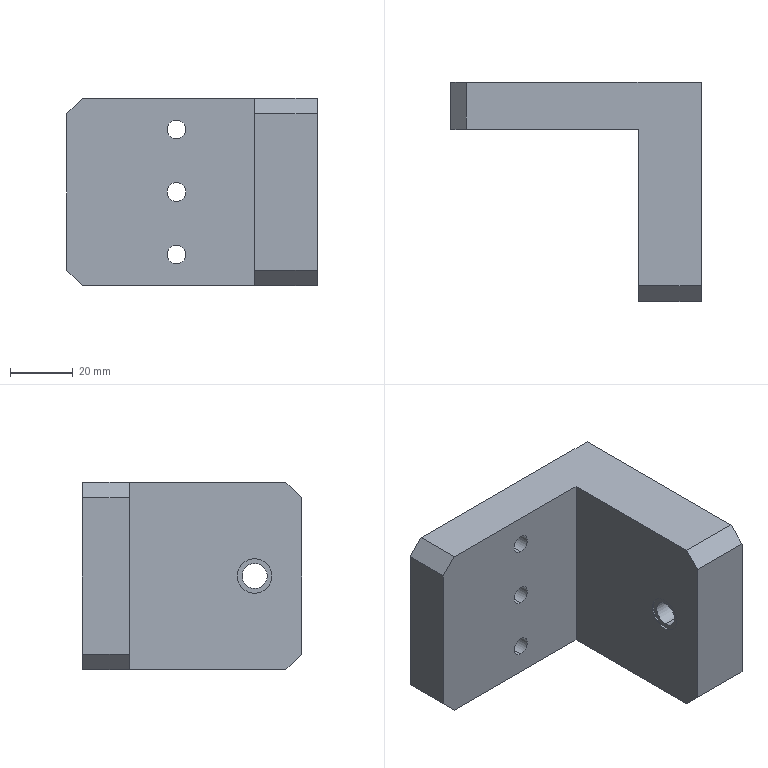Component | SolidWorks | ElectricalBoxAssembly2-1_AuxiliaryWheelFrame-1 | 1 solid | 23 faces | box 80 x 70 x 60 mm | volume 134825 mm3 | plane 13 | cylinder 10 | commonest cylinder face diameters 6 x6 11 x2 8 x2
build123d program:
from build123d import *

# Parameters (mm, degrees)
BOSS_EXTRUDE1_DEPTH           = 30
M8_TAPPED_HOLE1_D             = 8
SKETCH5_R                     = 2
CUT_EXTRUDE1_DEPTH            = 102.612
CHAMFER1_SIZE                 = 5
M6_TAPPED_HOLE2_D             = 6
M6_TAPPED_HOLE3_D             = 6
SKETCH1_R                     = 5.5
M8_SHOULDERSEAT_D11X0_5_DEPTH = 0.5


with BuildPart() as part:
    # Sketch1_2 → Boss-Extrude1 (new, symmetric)
    with BuildSketch(Plane.XY):
        Polygon((0, 0), (0, 70), (20, 70), (20, 15), (80, 15), (80, 0), align=None)
    extrude(amount=BOSS_EXTRUDE1_DEPTH, both=True)

    # M8 Tapped Hole1 (through all)
    with Locations(Plane(origin=(20, 0, 0), x_dir=(0, 0, -1), z_dir=(1, 0, 0))):
        with Locations((0, 55)):
            Hole(M8_TAPPED_HOLE1_D / 2)

    # Sketch5 → Cut-Extrude1 (cut, through all)
    with BuildSketch(Plane(origin=(0, 15, 0), x_dir=(1, 0, 0), z_dir=(0, 1, 0))):
        with Locations(Location((45, 20, 0), (0, 0, 270))):
            Circle(SKETCH5_R)
        with Locations(Location((45, -20, 0), (0, 0, 270))):
            Circle(SKETCH5_R)
        with Locations(Location((45, 0, 0), (0, 0, 270))):
            Circle(SKETCH5_R)
    extrude(amount=-CUT_EXTRUDE1_DEPTH, mode=Mode.SUBTRACT)

    # Chamfer1
    chamfer1_edges = [part.edges().sort_by_distance(p)[0] for p in [
        (10, 70, 30),
        (10, 70, -30),
        (80, 7.5, 30),
        (80, 7.5, -30),
    ]]
    chamfer(chamfer1_edges, length=CHAMFER1_SIZE)

    # M6 Tapped Hole2 (through all)
    with Locations(Plane(origin=(0, 15, 0), x_dir=(1, 0, 0), z_dir=(0, 1, 0))):
        with Locations((45, 20), (45, -20)):
            Hole(M6_TAPPED_HOLE2_D / 2)

    # M6 Tapped Hole3 (through all)
    with Locations(Plane(origin=(0, 15, 0), x_dir=(1, 0, 0), z_dir=(0, 1, 0))):
        with Locations((45, 0)):
            Hole(M6_TAPPED_HOLE3_D / 2)

    # Sketch1 → M8_ShoulderSeat_D11x0.5 (cut)
    with BuildSketch(Plane(origin=(20, 0, 0), x_dir=(0, 0, -1), z_dir=(1, 0, 0))):
        with Locations(Location((0, 55, 0), (0, 0, 90))):
            Circle(SKETCH1_R)
    extrude(amount=-M8_SHOULDERSEAT_D11X0_5_DEPTH, mode=Mode.SUBTRACT)


solid = part.part

# Placed as in the assembly
solid = solid.moved(Location((755.468, 389.666, 1526.399), (0, 0, 180)))
STEP:
#1=CARTESIAN_POINT('',(28.975,13.392,60.094));
#2=VERTEX_POINT('',#1);
#3=CARTESIAN_POINT('',(28.975,12.959,60.094));
#4=VERTEX_POINT('',#3);
#5=CARTESIAN_POINT('',(28.975,13.176,60.094));
#6=DIRECTION('',(-1.,-0.,-0.));
#7=DIRECTION('',(0.,-1.,0.));
#8=AXIS2_PLACEMENT_3D('',#5,#6,#7);
#9=CIRCLE('',#8,0.2165);
#10=EDGE_CURVE('',#2,#4,#9,.T.);
#11=ORIENTED_EDGE('',*,*,#10,.F.);
#12=CARTESIAN_POINT('',(28.955,13.392,60.094));
#13=VERTEX_POINT('',#12);
#14=CARTESIAN_POINT('',(28.975,13.392,60.094));
#15=DIRECTION('',(-1.,-0.,-0.));
#16=VECTOR('',#15,39.37);
#17=LINE('',#14,#16);
#18=EDGE_CURVE('',#2,#13,#17,.T.);
#19=ORIENTED_EDGE('',*,*,#18,.T.);
#20=CARTESIAN_POINT('',(28.955,12.959,60.094));
#21=VERTEX_POINT('',#20);
#22=CARTESIAN_POINT('',(28.955,13.176,60.094));
#23=DIRECTION('',(-1.,-0.,-0.));
#24=DIRECTION('',(0.,-1.,0.));
#25=AXIS2_PLACEMENT_3D('',#22,#23,#24);
#26=CIRCLE('',#25,0.2165);
#27=EDGE_CURVE('',#13,#21,#26,.T.);
#28=ORIENTED_EDGE('',*,*,#27,.T.);
#29=CARTESIAN_POINT('',(28.975,12.959,60.094));
#30=DIRECTION('',(-1.,-0.,-0.));
#31=VECTOR('',#30,39.37);
#32=LINE('',#29,#31);
#33=EDGE_CURVE('',#4,#21,#32,.T.);
#34=ORIENTED_EDGE('',*,*,#33,.F.);
#35=EDGE_LOOP('',(#11,#19,#28,#34));
#36=FACE_OUTER_BOUND('',#35,.T.);
#37=CARTESIAN_POINT('',(28.975,13.176,60.094));
#38=DIRECTION('',(-1.,-0.,-0.));
#39=DIRECTION('',(0.,-1.,0.));
#40=AXIS2_PLACEMENT_3D('',#37,#38,#39);
#41=CYLINDRICAL_SURFACE('',#40,0.2165);
#42=ADVANCED_FACE('',(#36),#41,.F.);
#43=CARTESIAN_POINT('',(27.971,15.341,59.976));
#44=VERTEX_POINT('',#43);
#45=CARTESIAN_POINT('',(27.971,15.341,60.213));
#46=VERTEX_POINT('',#45);
#47=CARTESIAN_POINT('',(27.971,15.341,60.094));
#48=DIRECTION('',(0.,-1.,-0.));
#49=DIRECTION('',(0.,0.,1.));
#50=AXIS2_PLACEMENT_3D('',#47,#48,#49);
#51=CIRCLE('',#50,0.1181);
#52=EDGE_CURVE('',#44,#46,#51,.T.);
#53=ORIENTED_EDGE('',*,*,#52,.F.);
#54=CARTESIAN_POINT('',(27.971,14.751,59.976));
#55=VERTEX_POINT('',#54);
#56=CARTESIAN_POINT('',(27.971,14.751,59.976));
#57=DIRECTION('',(0.,-1.,-0.));
#58=VECTOR('',#57,39.37);
#59=LINE('',#56,#58);
#60=EDGE_CURVE('',#44,#55,#59,.T.);
#61=ORIENTED_EDGE('',*,*,#60,.T.);
#62=CARTESIAN_POINT('',(27.971,14.751,60.213));
#63=VERTEX_POINT('',#62);
#64=CARTESIAN_POINT('',(27.971,14.751,60.094));
#65=DIRECTION('',(0.,-1.,-0.));
#66=DIRECTION('',(0.,0.,1.));
#67=AXIS2_PLACEMENT_3D('',#64,#65,#66);
#68=CIRCLE('',#67,0.1181);
#69=EDGE_CURVE('',#55,#63,#68,.T.);
#70=ORIENTED_EDGE('',*,*,#69,.T.);
#71=CARTESIAN_POINT('',(27.971,14.751,60.213));
#72=DIRECTION('',(0.,-1.,-0.));
#73=VECTOR('',#72,39.37);
#74=LINE('',#71,#73);
#75=EDGE_CURVE('',#46,#63,#74,.T.);
#76=ORIENTED_EDGE('',*,*,#75,.F.);
#77=EDGE_LOOP('',(#53,#61,#70,#76));
#78=FACE_OUTER_BOUND('',#77,.T.);
#79=CARTESIAN_POINT('',(27.971,14.751,60.094));
#80=DIRECTION('',(0.,-1.,-0.));
#81=DIRECTION('',(0.,0.,1.));
#82=AXIS2_PLACEMENT_3D('',#79,#80,#81);
#83=CYLINDRICAL_SURFACE('',#82,0.1181);
#84=ADVANCED_FACE('',(#78),#83,.F.);
#85=CARTESIAN_POINT('',(27.971,15.341,59.189));
#86=VERTEX_POINT('',#85);
#87=CARTESIAN_POINT('',(27.971,15.341,59.425));
#88=VERTEX_POINT('',#87);
#89=CARTESIAN_POINT('',(27.971,15.341,59.307));
#90=DIRECTION('',(0.,-1.,-0.));
#91=DIRECTION('',(0.,0.,1.));
#92=AXIS2_PLACEMENT_3D('',#89,#90,#91);
#93=CIRCLE('',#92,0.1181);
#94=EDGE_CURVE('',#86,#88,#93,.T.);
#95=ORIENTED_EDGE('',*,*,#94,.F.);
#96=CARTESIAN_POINT('',(27.971,14.751,59.189));
#97=VERTEX_POINT('',#96);
#98=CARTESIAN_POINT('',(27.971,14.751,59.189));
#99=DIRECTION('',(0.,-1.,-0.));
#100=VECTOR('',#99,39.37);
#101=LINE('',#98,#100);
#102=EDGE_CURVE('',#86,#97,#101,.T.);
#103=ORIENTED_EDGE('',*,*,#102,.T.);
#104=CARTESIAN_POINT('',(27.971,14.751,59.425));
#105=VERTEX_POINT('',#104);
#106=CARTESIAN_POINT('',(27.971,14.751,59.307));
#107=DIRECTION('',(0.,-1.,-0.));
#108=DIRECTION('',(0.,0.,1.));
#109=AXIS2_PLACEMENT_3D('',#106,#107,#108);
#110=CIRCLE('',#109,0.1181);
#111=EDGE_CURVE('',#97,#105,#110,.T.);
#112=ORIENTED_EDGE('',*,*,#111,.T.);
#113=CARTESIAN_POINT('',(27.971,14.751,59.425));
#114=DIRECTION('',(0.,-1.,-0.));
#115=VECTOR('',#114,39.37);
#116=LINE('',#113,#115);
#117=EDGE_CURVE('',#88,#105,#116,.T.);
#118=ORIENTED_EDGE('',*,*,#117,.F.);
#119=EDGE_LOOP('',(#95,#103,#112,#118));
#120=FACE_OUTER_BOUND('',#119,.T.);
#121=CARTESIAN_POINT('',(27.971,14.751,59.307));
#122=DIRECTION('',(0.,-1.,-0.));
#123=DIRECTION('',(0.,0.,1.));
#124=AXIS2_PLACEMENT_3D('',#121,#122,#123);
#125=CYLINDRICAL_SURFACE('',#124,0.1181);
#126=ADVANCED_FACE('',(#120),#125,.F.);
#127=CARTESIAN_POINT('',(27.971,15.341,60.764));
#128=VERTEX_POINT('',#127);
#129=CARTESIAN_POINT('',(27.971,15.341,61.));
#130=VERTEX_POINT('',#129);
#131=CARTESIAN_POINT('',(27.971,15.341,60.882));
#132=DIRECTION('',(0.,-1.,-0.));
#133=DIRECTION('',(0.,0.,1.));
#134=AXIS2_PLACEMENT_3D('',#131,#132,#133);
#135=CIRCLE('',#134,0.1181);
#136=EDGE_CURVE('',#128,#130,#135,.T.);
#137=ORIENTED_EDGE('',*,*,#136,.F.);
#138=CARTESIAN_POINT('',(27.971,14.751,60.764));
#139=VERTEX_POINT('',#138);
#140=CARTESIAN_POINT('',(27.971,14.751,60.764));
#141=DIRECTION('',(0.,-1.,-0.));
#142=VECTOR('',#141,39.37);
#143=LINE('',#140,#142);
#144=EDGE_CURVE('',#128,#139,#143,.T.);
#145=ORIENTED_EDGE('',*,*,#144,.T.);
#146=CARTESIAN_POINT('',(27.971,14.751,61.));
#147=VERTEX_POINT('',#146);
#148=CARTESIAN_POINT('',(27.971,14.751,60.882));
#149=DIRECTION('',(0.,-1.,-0.));
#150=DIRECTION('',(0.,0.,1.));
#151=AXIS2_PLACEMENT_3D('',#148,#149,#150);
#152=CIRCLE('',#151,0.1181);
#153=EDGE_CURVE('',#139,#147,#152,.T.);
#154=ORIENTED_EDGE('',*,*,#153,.T.);
#155=CARTESIAN_POINT('',(27.971,14.751,61.));
#156=DIRECTION('',(0.,-1.,-0.));
#157=VECTOR('',#156,39.37);
#158=LINE('',#155,#157);
#159=EDGE_CURVE('',#130,#147,#158,.T.);
#160=ORIENTED_EDGE('',*,*,#159,.F.);
#161=EDGE_LOOP('',(#137,#145,#154,#160));
#162=FACE_OUTER_BOUND('',#161,.T.);
#163=CARTESIAN_POINT('',(27.971,14.751,60.882));
#164=DIRECTION('',(0.,-1.,-0.));
#165=DIRECTION('',(0.,0.,1.));
#166=AXIS2_PLACEMENT_3D('',#163,#164,#165);
#167=CYLINDRICAL_SURFACE('',#166,0.1181);
#168=ADVANCED_FACE('',(#162),#167,.F.);
#169=CARTESIAN_POINT('',(29.743,13.176,60.252));
#170=VERTEX_POINT('',#169);
#171=CARTESIAN_POINT('',(29.743,13.176,59.937));
#172=VERTEX_POINT('',#171);
#173=CARTESIAN_POINT('',(29.743,13.176,60.094));
#174=DIRECTION('',(-1.,-0.,-0.));
#175=DIRECTION('',(0.,0.,-1.));
#176=AXIS2_PLACEMENT_3D('',#173,#174,#175);
#177=CIRCLE('',#176,0.1575);
#178=EDGE_CURVE('',#170,#172,#177,.T.);
#179=ORIENTED_EDGE('',*,*,#178,.F.);
#180=CARTESIAN_POINT('',(28.975,13.176,60.252));
#181=VERTEX_POINT('',#180);
#182=CARTESIAN_POINT('',(28.955,13.176,60.252));
#183=DIRECTION('',(-1.,-0.,-0.));
#184=VECTOR('',#183,39.37);
#185=LINE('',#182,#184);
#186=EDGE_CURVE('',#170,#181,#185,.T.);
#187=ORIENTED_EDGE('',*,*,#186,.T.);
#188=CARTESIAN_POINT('',(28.975,13.176,59.937));
#189=VERTEX_POINT('',#188);
#190=CARTESIAN_POINT('',(28.975,13.176,60.094));
#191=DIRECTION('',(1.,0.,0.));
#192=DIRECTION('',(0.,-1.,0.));
#193=AXIS2_PLACEMENT_3D('',#190,#191,#192);
#194=CIRCLE('',#193,0.1575);
#195=EDGE_CURVE('',#189,#181,#194,.T.);
#196=ORIENTED_EDGE('',*,*,#195,.F.);
#197=CARTESIAN_POINT('',(28.955,13.176,59.937));
#198=DIRECTION('',(-1.,-0.,-0.));
#199=VECTOR('',#198,39.37);
#200=LINE('',#197,#199);
#201=EDGE_CURVE('',#172,#189,#200,.T.);
#202=ORIENTED_EDGE('',*,*,#201,.F.);
#203=EDGE_LOOP('',(#179,#187,#196,#202));
#204=FACE_OUTER_BOUND('',#203,.T.);
#205=CARTESIAN_POINT('',(28.955,13.176,60.094));
#206=DIRECTION('',(-1.,-0.,-0.));
#207=DIRECTION('',(0.,0.,-1.));
#208=AXIS2_PLACEMENT_3D('',#205,#206,#207);
#209=CYLINDRICAL_SURFACE('',#208,0.1575);
#210=ADVANCED_FACE('',(#204),#209,.F.);
#211=ORIENTED_EDGE('',*,*,#186,.F.);
#212=CARTESIAN_POINT('',(29.743,13.176,60.094));
#213=DIRECTION('',(-1.,-0.,-0.));
#214=DIRECTION('',(0.,0.,-1.));
#215=AXIS2_PLACEMENT_3D('',#212,#213,#214);
#216=CIRCLE('',#215,0.1575);
#217=EDGE_CURVE('',#172,#170,#216,.T.);
#218=ORIENTED_EDGE('',*,*,#217,.F.);
#219=ORIENTED_EDGE('',*,*,#201,.T.);
#220=CARTESIAN_POINT('',(28.975,13.176,60.094));
#221=DIRECTION('',(1.,0.,0.));
#222=DIRECTION('',(0.,-1.,0.));
#223=AXIS2_PLACEMENT_3D('',#220,#221,#222);
#224=CIRCLE('',#223,0.1575);
#225=EDGE_CURVE('',#181,#189,#224,.T.);
#226=ORIENTED_EDGE('',*,*,#225,.F.);
#227=EDGE_LOOP('',(#211,#218,#219,#226));
#228=FACE_OUTER_BOUND('',#227,.T.);
#229=CARTESIAN_POINT('',(28.955,13.176,60.094));
#230=DIRECTION('',(-1.,-0.,-0.));
#231=DIRECTION('',(0.,0.,-1.));
#232=AXIS2_PLACEMENT_3D('',#229,#230,#231);
#233=CYLINDRICAL_SURFACE('',#232,0.1575);
#234=ADVANCED_FACE('',(#228),#233,.F.);
#235=CARTESIAN_POINT('',(27.971,15.341,60.094));
#236=DIRECTION('',(0.,-1.,-0.));
#237=DIRECTION('',(0.,0.,1.));
#238=AXIS2_PLACEMENT_3D('',#235,#236,#237);
#239=CIRCLE('',#238,0.1181);
#240=EDGE_CURVE('',#46,#44,#239,.T.);
#241=ORIENTED_EDGE('',*,*,#240,.T.);
#242=ORIENTED_EDGE('',*,*,#52,.T.);
#243=EDGE_LOOP('',(#241,#242));
#244=FACE_BOUND('',#243,.T.);
#245=CARTESIAN_POINT('',(27.971,15.341,59.307));
#246=DIRECTION('',(0.,-1.,-0.));
#247=DIRECTION('',(0.,0.,1.));
#248=AXIS2_PLACEMENT_3D('',#245,#246,#247);
#249=CIRCLE('',#248,0.1181);
#250=EDGE_CURVE('',#88,#86,#249,.T.);
#251=ORIENTED_EDGE('',*,*,#250,.T.);
#252=ORIENTED_EDGE('',*,*,#94,.T.);
#253=EDGE_LOOP('',(#251,#252));
#254=FACE_BOUND('',#253,.T.);
#255=CARTESIAN_POINT('',(27.971,15.341,60.882));
#256=DIRECTION('',(0.,-1.,-0.));
#257=DIRECTION('',(0.,0.,1.));
#258=AXIS2_PLACEMENT_3D('',#255,#256,#257);
#259=CIRCLE('',#258,0.1181);
#260=EDGE_CURVE('',#130,#128,#259,.T.);
#261=ORIENTED_EDGE('',*,*,#260,.T.);
#262=ORIENTED_EDGE('',*,*,#136,.T.);
#263=EDGE_LOOP('',(#261,#262));
#264=FACE_BOUND('',#263,.T.);
#265=CARTESIAN_POINT('',(29.743,15.341,58.913));
#266=VERTEX_POINT('',#265);
#267=CARTESIAN_POINT('',(26.79,15.341,58.913));
#268=VERTEX_POINT('',#267);
#269=CARTESIAN_POINT('',(26.593,15.341,58.913));
#270=DIRECTION('',(-1.,0.,-0.));
#271=VECTOR('',#270,39.37);
#272=LINE('',#269,#271);
#273=EDGE_CURVE('',#266,#268,#272,.T.);
#274=ORIENTED_EDGE('',*,*,#273,.T.);
#275=CARTESIAN_POINT('',(26.593,15.341,59.11));
#276=VERTEX_POINT('',#275);
#277=CARTESIAN_POINT('',(26.593,15.341,59.11));
#278=DIRECTION('',(-0.7071,0.,0.7071));
#279=VECTOR('',#278,39.37);
#280=LINE('',#277,#279);
#281=EDGE_CURVE('',#268,#276,#280,.T.);
#282=ORIENTED_EDGE('',*,*,#281,.T.);
#283=CARTESIAN_POINT('',(26.593,15.341,61.079));
#284=VERTEX_POINT('',#283);
#285=CARTESIAN_POINT('',(26.593,15.341,61.276));
#286=DIRECTION('',(0.,0.,-1.));
#287=VECTOR('',#286,39.37);
#288=LINE('',#285,#287);
#289=EDGE_CURVE('',#284,#276,#288,.T.);
#290=ORIENTED_EDGE('',*,*,#289,.F.);
#291=CARTESIAN_POINT('',(26.79,15.341,61.276));
#292=VERTEX_POINT('',#291);
#293=CARTESIAN_POINT('',(26.79,15.341,61.276));
#294=DIRECTION('',(0.7071,-0.,0.7071));
#295=VECTOR('',#294,39.37);
#296=LINE('',#293,#295);
#297=EDGE_CURVE('',#284,#292,#296,.T.);
#298=ORIENTED_EDGE('',*,*,#297,.T.);
#299=CARTESIAN_POINT('',(29.743,15.341,61.276));
#300=VERTEX_POINT('',#299);
#301=CARTESIAN_POINT('',(26.593,15.341,61.276));
#302=DIRECTION('',(-1.,0.,-0.));
#303=VECTOR('',#302,39.37);
#304=LINE('',#301,#303);
#305=EDGE_CURVE('',#300,#292,#304,.T.);
#306=ORIENTED_EDGE('',*,*,#305,.F.);
#307=CARTESIAN_POINT('',(29.743,15.341,61.276));
#308=DIRECTION('',(0.,0.,-1.));
#309=VECTOR('',#308,39.37);
#310=LINE('',#307,#309);
#311=EDGE_CURVE('',#300,#266,#310,.T.);
#312=ORIENTED_EDGE('',*,*,#311,.T.);
#313=EDGE_LOOP('',(#274,#282,#290,#298,#306,#312));
#314=FACE_OUTER_BOUND('',#313,.T.);
#315=CARTESIAN_POINT('',(26.593,15.341,61.276));
#316=DIRECTION('',(-0.,-1.,-0.));
#317=DIRECTION('',(1.,-0.,0.));
#318=AXIS2_PLACEMENT_3D('',#315,#316,#317);
#319=PLANE('',#318);
#320=ADVANCED_FACE('',(#244,#254,#264,#314),#319,.F.);
#321=ORIENTED_EDGE('',*,*,#289,.T.);
#322=CARTESIAN_POINT('',(26.593,14.751,59.11));
#323=VERTEX_POINT('',#322);
#324=CARTESIAN_POINT('',(26.593,14.751,59.11));
#325=DIRECTION('',(0.,-1.,-0.));
#326=VECTOR('',#325,39.37);
#327=LINE('',#324,#326);
#328=EDGE_CURVE('',#276,#323,#327,.T.);
#329=ORIENTED_EDGE('',*,*,#328,.T.);
#330=CARTESIAN_POINT('',(26.593,14.751,61.079));
#331=VERTEX_POINT('',#330);
#332=CARTESIAN_POINT('',(26.593,14.751,61.276));
#333=DIRECTION('',(0.,0.,-1.));
#334=VECTOR('',#333,39.37);
#335=LINE('',#332,#334);
#336=EDGE_CURVE('',#331,#323,#335,.T.);
#337=ORIENTED_EDGE('',*,*,#336,.F.);
#338=CARTESIAN_POINT('',(26.593,14.751,61.079));
#339=DIRECTION('',(-0.,1.,0.));
#340=VECTOR('',#339,39.37);
#341=LINE('',#338,#340);
#342=EDGE_CURVE('',#331,#284,#341,.T.);
#343=ORIENTED_EDGE('',*,*,#342,.T.);
#344=EDGE_LOOP('',(#321,#329,#337,#343));
#345=FACE_OUTER_BOUND('',#344,.T.);
#346=CARTESIAN_POINT('',(26.593,14.751,61.276));
#347=DIRECTION('',(1.,0.,0.));
#348=DIRECTION('',(-0.,-0.,1.));
#349=AXIS2_PLACEMENT_3D('',#346,#347,#348);
#350=PLANE('',#349);
#351=ADVANCED_FACE('',(#345),#350,.F.);
#352=CARTESIAN_POINT('',(27.971,14.751,60.094));
#353=DIRECTION('',(0.,-1.,-0.));
#354=DIRECTION('',(0.,0.,1.));
#355=AXIS2_PLACEMENT_3D('',#352,#353,#354);
#356=CIRCLE('',#355,0.1181);
#357=EDGE_CURVE('',#63,#55,#356,.T.);
#358=ORIENTED_EDGE('',*,*,#357,.F.);
#359=ORIENTED_EDGE('',*,*,#69,.F.);
#360=EDGE_LOOP('',(#358,#359));
#361=FACE_BOUND('',#360,.T.);
#362=CARTESIAN_POINT('',(27.971,14.751,59.307));
#363=DIRECTION('',(0.,-1.,-0.));
#364=DIRECTION('',(0.,0.,1.));
#365=AXIS2_PLACEMENT_3D('',#362,#363,#364);
#366=CIRCLE('',#365,0.1181);
#367=EDGE_CURVE('',#105,#97,#366,.T.);
#368=ORIENTED_EDGE('',*,*,#367,.F.);
#369=ORIENTED_EDGE('',*,*,#111,.F.);
#370=EDGE_LOOP('',(#368,#369));
#371=FACE_BOUND('',#370,.T.);
#372=CARTESIAN_POINT('',(27.971,14.751,60.882));
#373=DIRECTION('',(0.,-1.,-0.));
#374=DIRECTION('',(0.,0.,1.));
#375=AXIS2_PLACEMENT_3D('',#372,#373,#374);
#376=CIRCLE('',#375,0.1181);
#377=EDGE_CURVE('',#147,#139,#376,.T.);
#378=ORIENTED_EDGE('',*,*,#377,.F.);
#379=ORIENTED_EDGE('',*,*,#153,.F.);
#380=EDGE_LOOP('',(#378,#379));
#381=FACE_BOUND('',#380,.T.);
#382=ORIENTED_EDGE('',*,*,#336,.T.);
#383=CARTESIAN_POINT('',(26.79,14.751,58.913));
#384=VERTEX_POINT('',#383);
#385=CARTESIAN_POINT('',(26.593,14.751,59.11));
#386=DIRECTION('',(0.7071,-0.,-0.7071));
#387=VECTOR('',#386,39.37);
#388=LINE('',#385,#387);
#389=EDGE_CURVE('',#323,#384,#388,.T.);
#390=ORIENTED_EDGE('',*,*,#389,.T.);
#391=CARTESIAN_POINT('',(28.955,14.751,58.913));
#392=VERTEX_POINT('',#391);
#393=CARTESIAN_POINT('',(28.955,14.751,58.913));
#394=DIRECTION('',(1.,-0.,0.));
#395=VECTOR('',#394,39.37);
#396=LINE('',#393,#395);
#397=EDGE_CURVE('',#384,#392,#396,.T.);
#398=ORIENTED_EDGE('',*,*,#397,.T.);
#399=CARTESIAN_POINT('',(28.955,14.751,61.276));
#400=VERTEX_POINT('',#399);
#401=CARTESIAN_POINT('',(28.955,14.751,61.276));
#402=DIRECTION('',(0.,0.,-1.));
#403=VECTOR('',#402,39.37);
#404=LINE('',#401,#403);
#405=EDGE_CURVE('',#400,#392,#404,.T.);
#406=ORIENTED_EDGE('',*,*,#405,.F.);
#407=CARTESIAN_POINT('',(26.79,14.751,61.276));
#408=VERTEX_POINT('',#407);
#409=CARTESIAN_POINT('',(28.955,14.751,61.276));
#410=DIRECTION('',(1.,-0.,0.));
#411=VECTOR('',#410,39.37);
#412=LINE('',#409,#411);
#413=EDGE_CURVE('',#408,#400,#412,.T.);
#414=ORIENTED_EDGE('',*,*,#413,.F.);
#415=CARTESIAN_POINT('',(26.79,14.751,61.276));
#416=DIRECTION('',(-0.7071,0.,-0.7071));
#417=VECTOR('',#416,39.37);
#418=LINE('',#415,#417);
#419=EDGE_CURVE('',#408,#331,#418,.T.);
#420=ORIENTED_EDGE('',*,*,#419,.T.);
#421=EDGE_LOOP('',(#382,#390,#398,#406,#414,#420));
#422=FACE_OUTER_BOUND('',#421,.T.);
#423=CARTESIAN_POINT('',(28.955,14.751,61.276));
#424=DIRECTION('',(0.,1.,0.));
#425=DIRECTION('',(-1.,0.,-0.));
#426=AXIS2_PLACEMENT_3D('',#423,#424,#425);
#427=PLANE('',#426);
#428=ADVANCED_FACE('',(#361,#371,#381,#422),#427,.F.);
#429=CARTESIAN_POINT('',(28.955,13.176,60.094));
#430=DIRECTION('',(-1.,-0.,-0.));
#431=DIRECTION('',(0.,-1.,0.));
#432=AXIS2_PLACEMENT_3D('',#429,#430,#431);
#433=CIRCLE('',#432,0.2165);
#434=EDGE_CURVE('',#21,#13,#433,.T.);
#435=ORIENTED_EDGE('',*,*,#434,.F.);
#436=ORIENTED_EDGE('',*,*,#27,.F.);
#437=EDGE_LOOP('',(#435,#436));
#438=FACE_BOUND('',#437,.T.);
#439=CARTESIAN_POINT('',(28.955,12.782,58.913));
#440=VERTEX_POINT('',#439);
#441=CARTESIAN_POINT('',(28.955,12.585,58.913));
#442=DIRECTION('',(0.,-1.,-0.));
#443=VECTOR('',#442,39.37);
#444=LINE('',#441,#443);
#445=EDGE_CURVE('',#392,#440,#444,.T.);
#446=ORIENTED_EDGE('',*,*,#445,.T.);
#447=CARTESIAN_POINT('',(28.955,12.585,59.11));
#448=VERTEX_POINT('',#447);
#449=CARTESIAN_POINT('',(28.955,12.585,59.11));
#450=DIRECTION('',(-0.,-0.7071,0.7071));
#451=VECTOR('',#450,39.37);
#452=LINE('',#449,#451);
#453=EDGE_CURVE('',#440,#448,#452,.T.);
#454=ORIENTED_EDGE('',*,*,#453,.T.);
#455=CARTESIAN_POINT('',(28.955,12.585,61.079));
#456=VERTEX_POINT('',#455);
#457=CARTESIAN_POINT('',(28.955,12.585,61.276));
#458=DIRECTION('',(0.,0.,-1.));
#459=VECTOR('',#458,39.37);
#460=LINE('',#457,#459);
#461=EDGE_CURVE('',#456,#448,#460,.T.);
#462=ORIENTED_EDGE('',*,*,#461,.F.);
#463=CARTESIAN_POINT('',(28.955,12.782,61.276));
#464=VERTEX_POINT('',#463);
#465=CARTESIAN_POINT('',(28.955,12.782,61.276));
#466=DIRECTION('',(-0.,0.7071,0.7071));
#467=VECTOR('',#466,39.37);
#468=LINE('',#465,#467);
#469=EDGE_CURVE('',#456,#464,#468,.T.);
#470=ORIENTED_EDGE('',*,*,#469,.T.);
#471=CARTESIAN_POINT('',(28.955,12.585,61.276));
#472=DIRECTION('',(0.,-1.,-0.));
#473=VECTOR('',#472,39.37);
#474=LINE('',#471,#473);
#475=EDGE_CURVE('',#400,#464,#474,.T.);
#476=ORIENTED_EDGE('',*,*,#475,.F.);
#477=ORIENTED_EDGE('',*,*,#405,.T.);
#478=EDGE_LOOP('',(#446,#454,#462,#470,#476,#477));
#479=FACE_OUTER_BOUND('',#478,.T.);
#480=CARTESIAN_POINT('',(28.955,12.585,61.276));
#481=DIRECTION('',(1.,0.,0.));
#482=DIRECTION('',(-0.,1.,0.));
#483=AXIS2_PLACEMENT_3D('',#480,#481,#482);
#484=PLANE('',#483);
#485=ADVANCED_FACE('',(#438,#479),#484,.F.);
#486=ORIENTED_EDGE('',*,*,#461,.T.);
#487=CARTESIAN_POINT('',(29.743,12.585,59.11));
#488=VERTEX_POINT('',#487);
#489=CARTESIAN_POINT('',(29.743,12.585,59.11));
#490=DIRECTION('',(1.,0.,0.));
#491=VECTOR('',#490,39.37);
#492=LINE('',#489,#491);
#493=EDGE_CURVE('',#448,#488,#492,.T.);
#494=ORIENTED_EDGE('',*,*,#493,.T.);
#495=CARTESIAN_POINT('',(29.743,12.585,61.079));
#496=VERTEX_POINT('',#495);
#497=CARTESIAN_POINT('',(29.743,12.585,61.276));
#498=DIRECTION('',(0.,0.,-1.));
#499=VECTOR('',#498,39.37);
#500=LINE('',#497,#499);
#501=EDGE_CURVE('',#496,#488,#500,.T.);
#502=ORIENTED_EDGE('',*,*,#501,.F.);
#503=CARTESIAN_POINT('',(29.743,12.585,61.079));
#504=DIRECTION('',(-1.,-0.,-0.));
#505=VECTOR('',#504,39.37);
#506=LINE('',#503,#505);
#507=EDGE_CURVE('',#496,#456,#506,.T.);
#508=ORIENTED_EDGE('',*,*,#507,.T.);
#509=EDGE_LOOP('',(#486,#494,#502,#508));
#510=FACE_OUTER_BOUND('',#509,.T.);
#511=CARTESIAN_POINT('',(29.743,12.585,61.276));
#512=DIRECTION('',(-0.,1.,0.));
#513=DIRECTION('',(0.,0.,-1.));
#514=AXIS2_PLACEMENT_3D('',#511,#512,#513);
#515=PLANE('',#514);
#516=ADVANCED_FACE('',(#510),#515,.F.);
#517=ORIENTED_EDGE('',*,*,#217,.T.);
#518=ORIENTED_EDGE('',*,*,#178,.T.);
#519=EDGE_LOOP('',(#517,#518));
#520=FACE_BOUND('',#519,.T.);
#521=ORIENTED_EDGE('',*,*,#501,.T.);
#522=CARTESIAN_POINT('',(29.743,12.782,58.913));
#523=VERTEX_POINT('',#522);
#524=CARTESIAN_POINT('',(29.743,12.585,59.11));
#525=DIRECTION('',(0.,0.7071,-0.7071));
#526=VECTOR('',#525,39.37);
#527=LINE('',#524,#526);
#528=EDGE_CURVE('',#488,#523,#527,.T.);
#529=ORIENTED_EDGE('',*,*,#528,.T.);
#530=CARTESIAN_POINT('',(29.743,15.341,58.913));
#531=DIRECTION('',(-0.,1.,0.));
#532=VECTOR('',#531,39.37);
#533=LINE('',#530,#532);
#534=EDGE_CURVE('',#523,#266,#533,.T.);
#535=ORIENTED_EDGE('',*,*,#534,.T.);
#536=ORIENTED_EDGE('',*,*,#311,.F.);
#537=CARTESIAN_POINT('',(29.743,12.782,61.276));
#538=VERTEX_POINT('',#537);
#539=CARTESIAN_POINT('',(29.743,15.341,61.276));
#540=DIRECTION('',(-0.,1.,0.));
#541=VECTOR('',#540,39.37);
#542=LINE('',#539,#541);
#543=EDGE_CURVE('',#538,#300,#542,.T.);
#544=ORIENTED_EDGE('',*,*,#543,.F.);
#545=CARTESIAN_POINT('',(29.743,12.782,61.276));
#546=DIRECTION('',(0.,-0.7071,-0.7071));
#547=VECTOR('',#546,39.37);
#548=LINE('',#545,#547);
#549=EDGE_CURVE('',#538,#496,#548,.T.);
#550=ORIENTED_EDGE('',*,*,#549,.T.);
#551=EDGE_LOOP('',(#521,#529,#535,#536,#544,#550));
#552=FACE_OUTER_BOUND('',#551,.T.);
#553=CARTESIAN_POINT('',(29.743,15.341,61.276));
#554=DIRECTION('',(-1.,-0.,-0.));
#555=DIRECTION('',(0.,0.,-1.));
#556=AXIS2_PLACEMENT_3D('',#553,#554,#555);
#557=PLANE('',#556);
#558=ADVANCED_FACE('',(#520,#552),#557,.F.);
#559=ORIENTED_EDGE('',*,*,#305,.T.);
#560=CARTESIAN_POINT('',(26.79,15.341,61.276));
#561=DIRECTION('',(0.,-1.,-0.));
#562=VECTOR('',#561,39.37);
#563=LINE('',#560,#562);
#564=EDGE_CURVE('',#292,#408,#563,.T.);
#565=ORIENTED_EDGE('',*,*,#564,.T.);
#566=ORIENTED_EDGE('',*,*,#413,.T.);
#567=ORIENTED_EDGE('',*,*,#475,.T.);
#568=CARTESIAN_POINT('',(29.743,12.782,61.276));
#569=DIRECTION('',(1.,0.,0.));
#570=VECTOR('',#569,39.37);
#571=LINE('',#568,#570);
#572=EDGE_CURVE('',#464,#538,#571,.T.);
#573=ORIENTED_EDGE('',*,*,#572,.T.);
#574=ORIENTED_EDGE('',*,*,#543,.T.);
#575=EDGE_LOOP('',(#559,#565,#566,#567,#573,#574));
#576=FACE_OUTER_BOUND('',#575,.T.);
#577=CARTESIAN_POINT('',(29.743,15.341,61.276));
#578=DIRECTION('',(0.,0.,-1.));
#579=DIRECTION('',(1.,0.,0.));
#580=AXIS2_PLACEMENT_3D('',#577,#578,#579);
#581=PLANE('',#580);
#582=ADVANCED_FACE('',(#576),#581,.F.);
#583=ORIENTED_EDGE('',*,*,#397,.F.);
#584=CARTESIAN_POINT('',(26.79,15.341,58.913));
#585=DIRECTION('',(-0.,1.,0.));
#586=VECTOR('',#585,39.37);
#587=LINE('',#584,#586);
#588=EDGE_CURVE('',#384,#268,#587,.T.);
#589=ORIENTED_EDGE('',*,*,#588,.T.);
#590=ORIENTED_EDGE('',*,*,#273,.F.);
#591=ORIENTED_EDGE('',*,*,#534,.F.);
#592=CARTESIAN_POINT('',(28.955,12.782,58.913));
#593=DIRECTION('',(-1.,-0.,-0.));
#594=VECTOR('',#593,39.37);
#595=LINE('',#592,#594);
#596=EDGE_CURVE('',#523,#440,#595,.T.);
#597=ORIENTED_EDGE('',*,*,#596,.T.);
#598=ORIENTED_EDGE('',*,*,#445,.F.);
#599=EDGE_LOOP('',(#583,#589,#590,#591,#597,#598));
#600=FACE_OUTER_BOUND('',#599,.T.);
#601=CARTESIAN_POINT('',(29.743,15.341,58.913));
#602=DIRECTION('',(0.,0.,-1.));
#603=DIRECTION('',(1.,0.,0.));
#604=AXIS2_PLACEMENT_3D('',#601,#602,#603);
#605=PLANE('',#604);
#606=ADVANCED_FACE('',(#600),#605,.T.);
#607=ORIENTED_EDGE('',*,*,#281,.F.);
#608=ORIENTED_EDGE('',*,*,#588,.F.);
#609=ORIENTED_EDGE('',*,*,#389,.F.);
#610=ORIENTED_EDGE('',*,*,#328,.F.);
#611=EDGE_LOOP('',(#607,#608,#609,#610));
#612=FACE_OUTER_BOUND('',#611,.T.);
#613=CARTESIAN_POINT('',(26.593,14.751,59.11));
#614=DIRECTION('',(-0.7071,-0.,-0.7071));
#615=DIRECTION('',(-0.,1.,0.));
#616=AXIS2_PLACEMENT_3D('',#613,#614,#615);
#617=PLANE('',#616);
#618=ADVANCED_FACE('',(#612),#617,.T.);
#619=ORIENTED_EDGE('',*,*,#297,.F.);
#620=ORIENTED_EDGE('',*,*,#342,.F.);
#621=ORIENTED_EDGE('',*,*,#419,.F.);
#622=ORIENTED_EDGE('',*,*,#564,.F.);
#623=EDGE_LOOP('',(#619,#620,#621,#622));
#624=FACE_OUTER_BOUND('',#623,.T.);
#625=CARTESIAN_POINT('',(26.79,15.341,61.276));
#626=DIRECTION('',(0.7071,0.,-0.7071));
#627=DIRECTION('',(0.,-1.,-0.));
#628=AXIS2_PLACEMENT_3D('',#625,#626,#627);
#629=PLANE('',#628);
#630=ADVANCED_FACE('',(#624),#629,.F.);
#631=ORIENTED_EDGE('',*,*,#453,.F.);
#632=ORIENTED_EDGE('',*,*,#596,.F.);
#633=ORIENTED_EDGE('',*,*,#528,.F.);
#634=ORIENTED_EDGE('',*,*,#493,.F.);
#635=EDGE_LOOP('',(#631,#632,#633,#634));
#636=FACE_OUTER_BOUND('',#635,.T.);
#637=CARTESIAN_POINT('',(29.743,12.585,59.11));
#638=DIRECTION('',(0.,-0.7071,-0.7071));
#639=DIRECTION('',(-1.,-0.,-0.));
#640=AXIS2_PLACEMENT_3D('',#637,#638,#639);
#641=PLANE('',#640);
#642=ADVANCED_FACE('',(#636),#641,.T.);
#643=ORIENTED_EDGE('',*,*,#469,.F.);
#644=ORIENTED_EDGE('',*,*,#507,.F.);
#645=ORIENTED_EDGE('',*,*,#549,.F.);
#646=ORIENTED_EDGE('',*,*,#572,.F.);
#647=EDGE_LOOP('',(#643,#644,#645,#646));
#648=FACE_OUTER_BOUND('',#647,.T.);
#649=CARTESIAN_POINT('',(29.743,12.782,61.276));
#650=DIRECTION('',(0.,0.7071,-0.7071));
#651=DIRECTION('',(1.,0.,0.));
#652=AXIS2_PLACEMENT_3D('',#649,#650,#651);
#653=PLANE('',#652);
#654=ADVANCED_FACE('',(#648),#653,.F.);
#655=ORIENTED_EDGE('',*,*,#144,.F.);
#656=ORIENTED_EDGE('',*,*,#260,.F.);
#657=ORIENTED_EDGE('',*,*,#159,.T.);
#658=ORIENTED_EDGE('',*,*,#377,.T.);
#659=EDGE_LOOP('',(#655,#656,#657,#658));
#660=FACE_OUTER_BOUND('',#659,.T.);
#661=CARTESIAN_POINT('',(27.971,14.751,60.882));
#662=DIRECTION('',(0.,-1.,-0.));
#663=DIRECTION('',(0.,0.,1.));
#664=AXIS2_PLACEMENT_3D('',#661,#662,#663);
#665=CYLINDRICAL_SURFACE('',#664,0.1181);
#666=ADVANCED_FACE('',(#660),#665,.F.);
#667=ORIENTED_EDGE('',*,*,#102,.F.);
#668=ORIENTED_EDGE('',*,*,#250,.F.);
#669=ORIENTED_EDGE('',*,*,#117,.T.);
#670=ORIENTED_EDGE('',*,*,#367,.T.);
#671=EDGE_LOOP('',(#667,#668,#669,#670));
#672=FACE_OUTER_BOUND('',#671,.T.);
#673=CARTESIAN_POINT('',(27.971,14.751,59.307));
#674=DIRECTION('',(0.,-1.,-0.));
#675=DIRECTION('',(0.,0.,1.));
#676=AXIS2_PLACEMENT_3D('',#673,#674,#675);
#677=CYLINDRICAL_SURFACE('',#676,0.1181);
#678=ADVANCED_FACE('',(#672),#677,.F.);
#679=ORIENTED_EDGE('',*,*,#60,.F.);
#680=ORIENTED_EDGE('',*,*,#240,.F.);
#681=ORIENTED_EDGE('',*,*,#75,.T.);
#682=ORIENTED_EDGE('',*,*,#357,.T.);
#683=EDGE_LOOP('',(#679,#680,#681,#682));
#684=FACE_OUTER_BOUND('',#683,.T.);
#685=CARTESIAN_POINT('',(27.971,14.751,60.094));
#686=DIRECTION('',(0.,-1.,-0.));
#687=DIRECTION('',(0.,0.,1.));
#688=AXIS2_PLACEMENT_3D('',#685,#686,#687);
#689=CYLINDRICAL_SURFACE('',#688,0.1181);
#690=ADVANCED_FACE('',(#684),#689,.F.);
#691=CARTESIAN_POINT('',(28.975,13.176,60.094));
#692=DIRECTION('',(-1.,-0.,-0.));
#693=DIRECTION('',(0.,-1.,0.));
#694=AXIS2_PLACEMENT_3D('',#691,#692,#693);
#695=CIRCLE('',#694,0.2165);
#696=EDGE_CURVE('',#4,#2,#695,.T.);
#697=ORIENTED_EDGE('',*,*,#696,.T.);
#698=ORIENTED_EDGE('',*,*,#10,.T.);
#699=EDGE_LOOP('',(#697,#698));
#700=FACE_OUTER_BOUND('',#699,.T.);
#701=ORIENTED_EDGE('',*,*,#195,.T.);
#702=ORIENTED_EDGE('',*,*,#225,.T.);
#703=EDGE_LOOP('',(#701,#702));
#704=FACE_BOUND('',#703,.T.);
#705=CARTESIAN_POINT('',(28.975,13.176,60.094));
#706=DIRECTION('',(-1.,-0.,-0.));
#707=DIRECTION('',(0.,-1.,-0.));
#708=AXIS2_PLACEMENT_3D('',#705,#706,#707);
#709=PLANE('',#708);
#710=ADVANCED_FACE('',(#700,#704),#709,.T.);
#711=ORIENTED_EDGE('',*,*,#18,.F.);
#712=ORIENTED_EDGE('',*,*,#696,.F.);
#713=ORIENTED_EDGE('',*,*,#33,.T.);
#714=ORIENTED_EDGE('',*,*,#434,.T.);
#715=EDGE_LOOP('',(#711,#712,#713,#714));
#716=FACE_OUTER_BOUND('',#715,.T.);
#717=CARTESIAN_POINT('',(28.975,13.176,60.094));
#718=DIRECTION('',(-1.,-0.,-0.));
#719=DIRECTION('',(0.,-1.,0.));
#720=AXIS2_PLACEMENT_3D('',#717,#718,#719);
#721=CYLINDRICAL_SURFACE('',#720,0.2165);
#722=ADVANCED_FACE('',(#716),#721,.F.);
#723=CLOSED_SHELL('',(#42,#84,#126,#168,#210,#234,#320,#351,#428,#485,#516,#558,#582,#606,#618,#630,#642,#654,#666,#678,#690,#710,#722));
#724=MANIFOLD_SOLID_BREP('',#723);
#725=CARTESIAN_POINT('',(0.,0.,0.));
#726=DIRECTION('',(0.,0.,1.));
#727=DIRECTION('',(1.,0.,0.));
#728=AXIS2_PLACEMENT_3D('',#725,#726,#727);
#729=(LENGTH_UNIT()NAMED_UNIT(*)SI_UNIT($,.METRE.));
#730=LENGTH_MEASURE_WITH_UNIT(LENGTH_MEASURE(0.0254),#729);
#731=DIMENSIONAL_EXPONENTS(1.,0.,0.,0.,0.,0.,0.);
#732=(CONVERSION_BASED_UNIT('',#730)LENGTH_UNIT()NAMED_UNIT(#731));
#733=UNCERTAINTY_MEASURE_WITH_UNIT(LENGTH_MEASURE(0.00001),#732,'','');
#734=(NAMED_UNIT(*)PLANE_ANGLE_UNIT()SI_UNIT($,.RADIAN.));
#735=(NAMED_UNIT(*)SI_UNIT($,.STERADIAN.)SOLID_ANGLE_UNIT());
#736=(GEOMETRIC_REPRESENTATION_CONTEXT(3)GLOBAL_UNCERTAINTY_ASSIGNED_CONTEXT((#733))GLOBAL_UNIT_ASSIGNED_CONTEXT((#732,#734,#735))REPRESENTATION_CONTEXT('',''));
#737=ADVANCED_BREP_SHAPE_REPRESENTATION('',(#724,#728),#736);
#738=COLOUR_RGB('',0.7922,0.8196,0.9333);
#739=FILL_AREA_STYLE_COLOUR('',#738);
#740=FILL_AREA_STYLE('',(#739));
#741=SURFACE_STYLE_FILL_AREA(#740);
#742=SURFACE_SIDE_STYLE('',(#741));
#743=SURFACE_STYLE_USAGE(.BOTH.,#742);
#744=PRESENTATION_STYLE_ASSIGNMENT((#743));
#745=STYLED_ITEM('',(#744),#724);
#746=PRESENTATION_LAYER_ASSIGNMENT('','',(#745));
#747=(LENGTH_UNIT()NAMED_UNIT(*)SI_UNIT($,.METRE.));
#748=LENGTH_MEASURE_WITH_UNIT(LENGTH_MEASURE(0.0254),#747);
#749=DIMENSIONAL_EXPONENTS(1.,0.,0.,0.,0.,0.,0.);
#750=(CONVERSION_BASED_UNIT('',#748)LENGTH_UNIT()NAMED_UNIT(#749));
#751=UNCERTAINTY_MEASURE_WITH_UNIT(LENGTH_MEASURE(0.00001),#750,'','');
#752=(NAMED_UNIT(*)PLANE_ANGLE_UNIT()SI_UNIT($,.RADIAN.));
#753=(NAMED_UNIT(*)SI_UNIT($,.STERADIAN.)SOLID_ANGLE_UNIT());
#754=(GEOMETRIC_REPRESENTATION_CONTEXT(3)GLOBAL_UNCERTAINTY_ASSIGNED_CONTEXT((#751))GLOBAL_UNIT_ASSIGNED_CONTEXT((#750,#752,#753))REPRESENTATION_CONTEXT('',''));
#755=MECHANICAL_DESIGN_GEOMETRIC_PRESENTATION_REPRESENTATION('',(#745),#754);